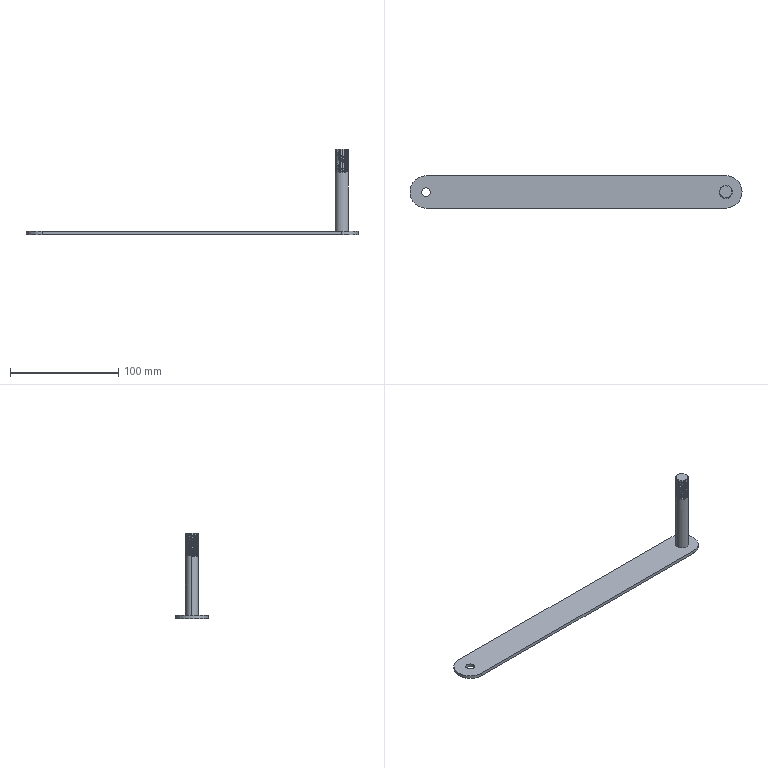Component | SolidWorks | M_LL_ KOL-1 | 1 solid | 62 faces | volume 35114 mm3 | cylinder 49 | plane 8 | spline 3 | cone 2 | commonest cylinder face diameters 12 x42 8 x4 30 x3